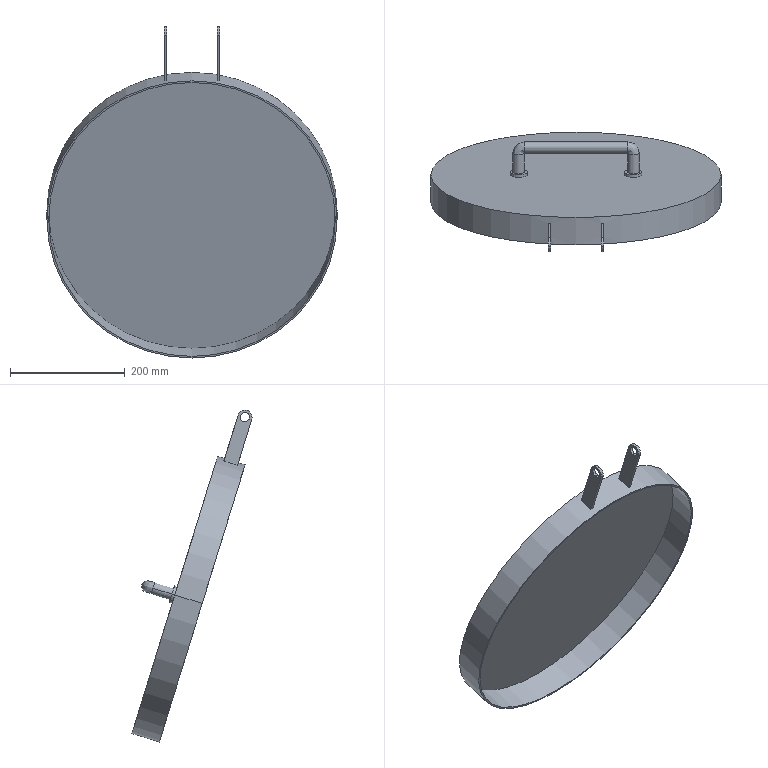Component | SolidWorks | Lid-2 | 1 solid | 45 faces | volume 943393 mm3 | cylinder 22 | plane 21 | spline 2 | commonest cylinder face diameters 20 x6 16 x4 30 x4 25 x4 506 x2 500 x2